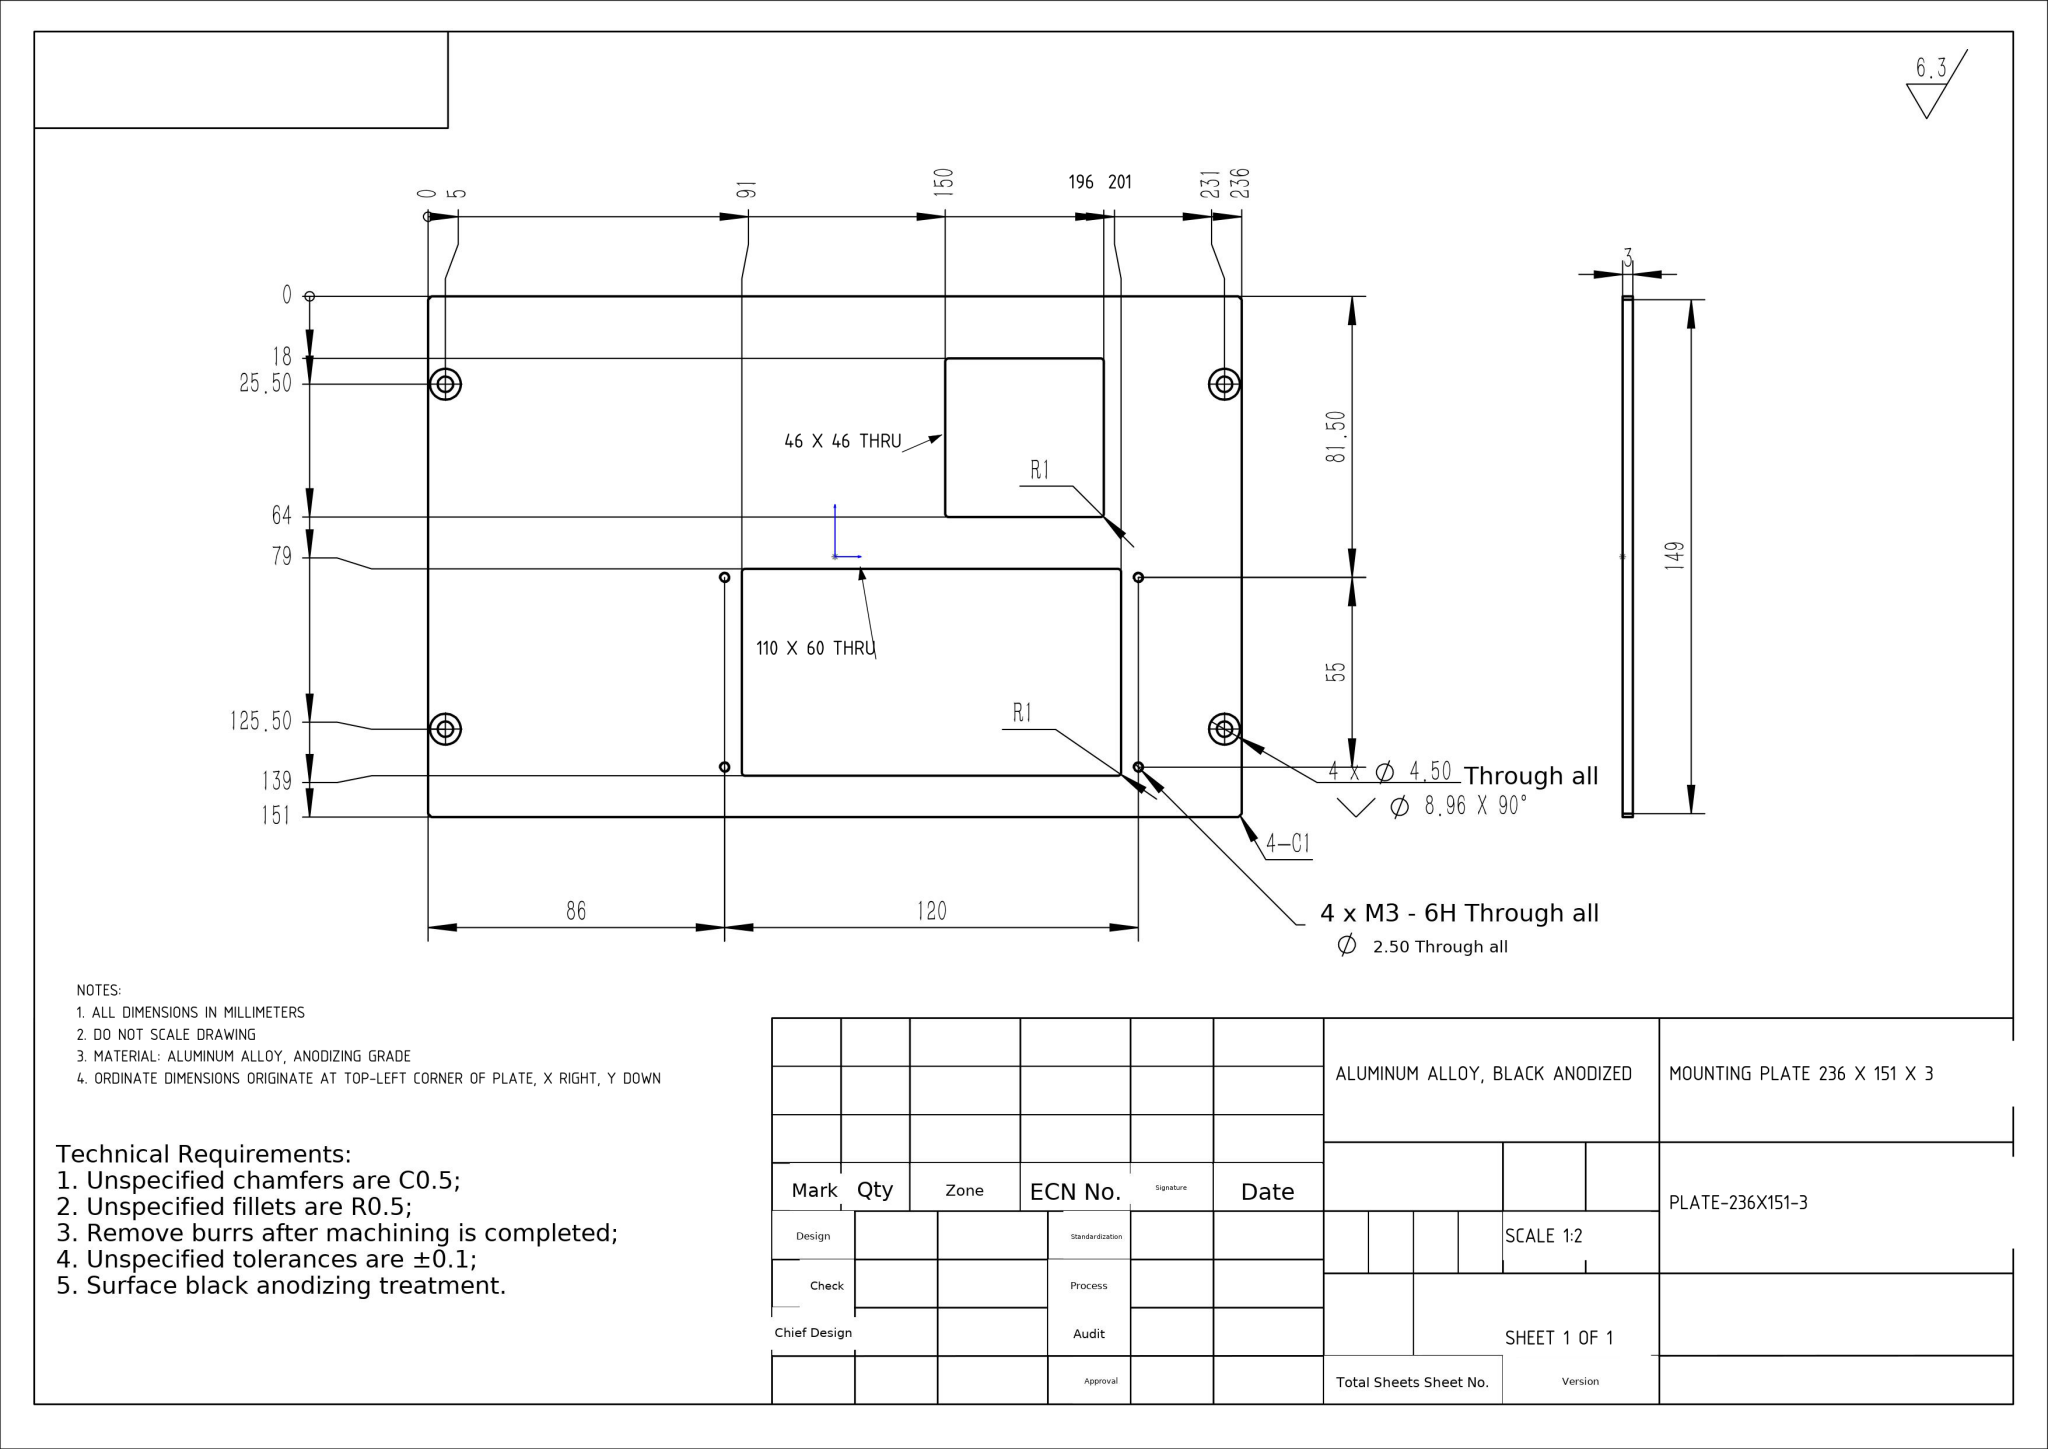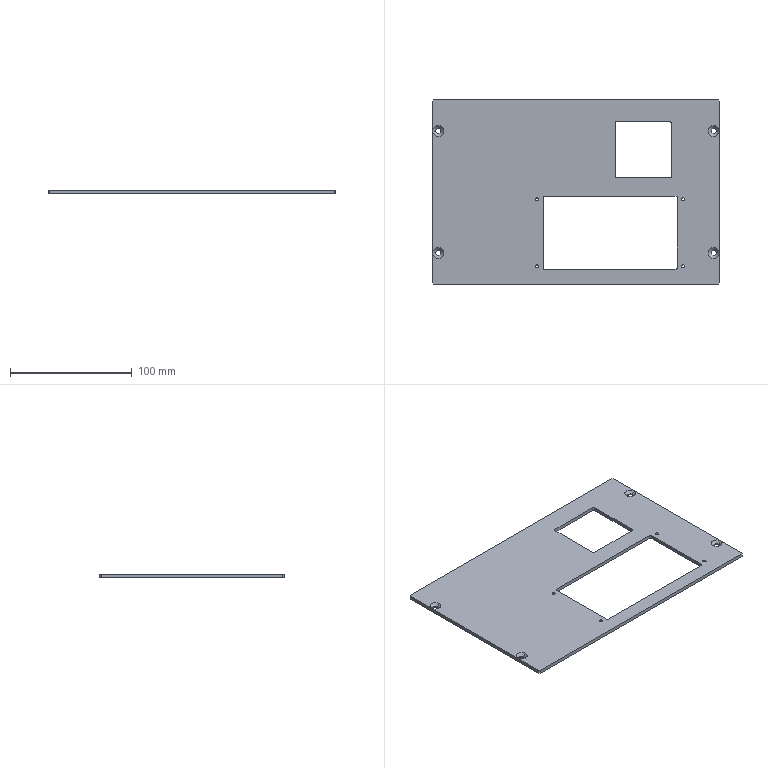Part | NX | mm | 1 solid | 50 faces | box 236 x 151 x 3 mm | volume 80322 mm3 | cylinder 24 | plane 18 | cone 8 | commonest cylinder face diameters 2.5 x8 4.5 x8 2 x8